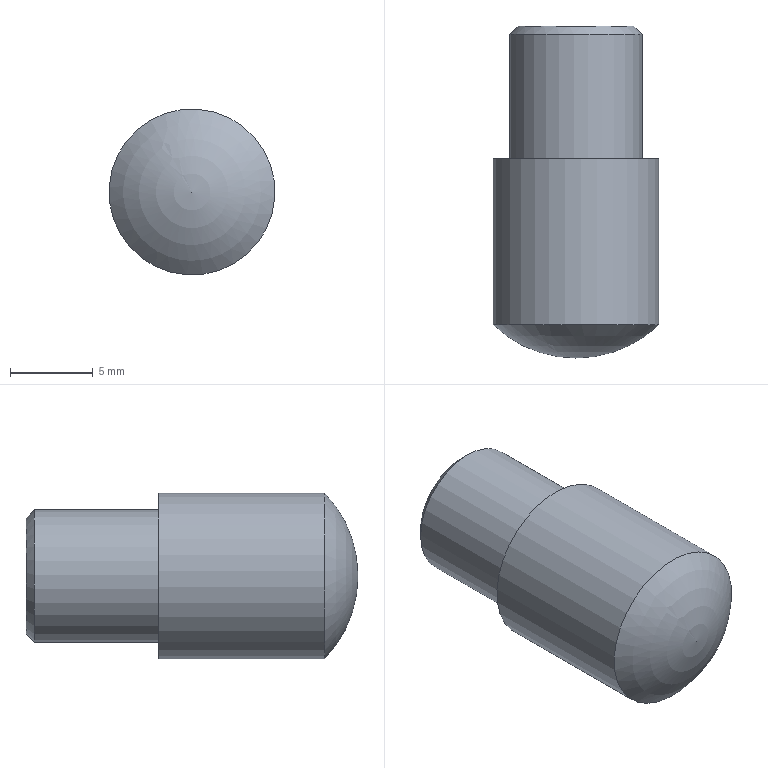Component | NX | 4_PIN | 1 solid | 6 faces | box 10 x 20 x 10 mm | volume 1267 mm3 | cylinder 2 | plane 2 | cone 1 | sphere 1 | commonest cylinder face diameters 10 x1 8 x1
STEP:
#1=CARTESIAN_POINT('',(0.,0.,0.));
#2=DIRECTION('',(0.,0.,1.));
#3=DIRECTION('',(1.,0.,0.));
#4=AXIS2_PLACEMENT_3D('',#1,#2,#3);
#5=CARTESIAN_POINT('',(6.35,16.63,-4.828));
#6=VERTEX_POINT('',#5);
#7=CARTESIAN_POINT('',(2.02,16.63,-7.328));
#8=DIRECTION('',(0.,-1.,0.));
#9=DIRECTION('',(0.866,0.,0.5));
#10=AXIS2_PLACEMENT_3D('',#7,#8,#9);
#11=CIRCLE('',#10,5.);
#12=CARTESIAN_POINT('',(2.02,4.63,-7.328));
#13=DIRECTION('',(0.,1.,0.));
#14=DIRECTION('',(0.866,0.,0.5));
#15=AXIS2_PLACEMENT_3D('',#12,#13,#14);
#16=CYLINDRICAL_SURFACE('',#15,5.);
#17=CARTESIAN_POINT('',(6.283,12.));
#18=DIRECTION('',(-1.,0.));
#19=VECTOR('',#18,1.);
#20=LINE('',#17,#19);
#21=(GEOMETRIC_REPRESENTATION_CONTEXT(2)PARAMETRIC_REPRESENTATION_CONTEXT()REPRESENTATION_CONTEXT('',''));
#22=DEFINITIONAL_REPRESENTATION('',(#20),#21);
#23=PCURVE('',#16,#22);
#24=CARTESIAN_POINT('',(2.02,16.63,-7.328));
#25=DIRECTION('',(0.,1.,0.));
#26=DIRECTION('',(0.866,0.,0.5));
#27=AXIS2_PLACEMENT_3D('',#24,#25,#26);
#28=PLANE('',#27);
#29=CARTESIAN_POINT('',(5.,0.));
#30=CARTESIAN_POINT('',(5.,-8.66));
#31=CARTESIAN_POINT('',(-2.5,-4.33));
#32=CARTESIAN_POINT('',(-10.,-0.));
#33=CARTESIAN_POINT('',(-2.5,4.33));
#34=CARTESIAN_POINT('',(5.,8.66));
#35=CARTESIAN_POINT('',(5.,0.));
#36=(BOUNDED_CURVE()B_SPLINE_CURVE(2,(#29,#30,#31,#32,#33,#34,#35),.UNSPECIFIED.,.T.,.F.)B_SPLINE_CURVE_WITH_KNOTS((1,2,2,2,2,1),(-2.094,0.,2.094,4.189,6.283,8.378),.UNSPECIFIED.)CURVE()GEOMETRIC_REPRESENTATION_ITEM()RATIONAL_B_SPLINE_CURVE((1.,0.5,1.,0.5,1.,0.5,1.))REPRESENTATION_ITEM(''));
#37=(GEOMETRIC_REPRESENTATION_CONTEXT(2)PARAMETRIC_REPRESENTATION_CONTEXT()REPRESENTATION_CONTEXT('',''));
#38=DEFINITIONAL_REPRESENTATION('',(#36),#37);
#39=PCURVE('',#28,#38);
#40=SURFACE_CURVE('',#11,(#23,#39),.PCURVE_S1.);
#41=EDGE_CURVE('',#6,#6,#40,.T.);
#42=ORIENTED_EDGE('',*,*,#41,.T.);
#43=CARTESIAN_POINT('',(6.35,6.63,-4.828));
#44=VERTEX_POINT('',#43);
#45=CARTESIAN_POINT('',(6.35,6.63,-4.828));
#46=CARTESIAN_POINT('',(6.35,16.63,-4.828));
#47=B_SPLINE_CURVE_WITH_KNOTS('',1,(#45,#46),.UNSPECIFIED.,.F.,.F.,(2,2),(2.,12.),.PIECEWISE_BEZIER_KNOTS.);
#48=CARTESIAN_POINT('',(0.,0.));
#49=DIRECTION('',(0.,1.));
#50=VECTOR('',#49,1.);
#51=LINE('',#48,#50);
#52=(GEOMETRIC_REPRESENTATION_CONTEXT(2)PARAMETRIC_REPRESENTATION_CONTEXT()REPRESENTATION_CONTEXT('',''));
#53=DEFINITIONAL_REPRESENTATION('',(#51),#52);
#54=PCURVE('',#16,#53);
#55=CARTESIAN_POINT('',(6.283,0.));
#56=DIRECTION('',(0.,1.));
#57=VECTOR('',#56,1.);
#58=LINE('',#55,#57);
#59=(GEOMETRIC_REPRESENTATION_CONTEXT(2)PARAMETRIC_REPRESENTATION_CONTEXT()REPRESENTATION_CONTEXT('',''));
#60=DEFINITIONAL_REPRESENTATION('',(#58),#59);
#61=PCURVE('',#16,#60);
#62=SEAM_CURVE('',#47,(#54,#61),.PCURVE_S1.);
#63=EDGE_CURVE('',#44,#6,#62,.T.);
#64=ORIENTED_EDGE('',*,*,#63,.F.);
#65=CARTESIAN_POINT('',(-0.4796,6.63,-2.998));
#66=VERTEX_POINT('',#65);
#67=CARTESIAN_POINT('',(2.02,6.63,-7.328));
#68=DIRECTION('',(0.,1.,0.));
#69=DIRECTION('',(0.866,0.,0.5));
#70=AXIS2_PLACEMENT_3D('',#67,#68,#69);
#71=CIRCLE('',#70,5.);
#72=CARTESIAN_POINT('',(0.,2.));
#73=DIRECTION('',(1.,0.));
#74=VECTOR('',#73,1.);
#75=LINE('',#72,#74);
#76=(GEOMETRIC_REPRESENTATION_CONTEXT(2)PARAMETRIC_REPRESENTATION_CONTEXT()REPRESENTATION_CONTEXT('',''));
#77=DEFINITIONAL_REPRESENTATION('',(#75),#76);
#78=PCURVE('',#16,#77);
#79=CARTESIAN_POINT('',(2.02,11.88,-7.328));
#80=DIRECTION('',(-0.,1.,0.));
#81=DIRECTION('',(-0.5,-0.,0.866));
#82=AXIS2_PLACEMENT_3D('',#79,#80,#81);
#83=SPHERICAL_SURFACE('',#82,7.25);
#84=CARTESIAN_POINT('',(1.571,-0.8098));
#85=CARTESIAN_POINT('',(1.666,-0.8098));
#86=CARTESIAN_POINT('',(1.856,-0.8098));
#87=CARTESIAN_POINT('',(2.142,-0.8098));
#88=CARTESIAN_POINT('',(2.428,-0.8098));
#89=CARTESIAN_POINT('',(2.713,-0.8098));
#90=CARTESIAN_POINT('',(2.999,-0.8098));
#91=CARTESIAN_POINT('',(3.284,-0.8098));
#92=CARTESIAN_POINT('',(3.57,-0.8098));
#93=CARTESIAN_POINT('',(3.856,-0.8098));
#94=CARTESIAN_POINT('',(4.141,-0.8098));
#95=CARTESIAN_POINT('',(4.427,-0.8098));
#96=CARTESIAN_POINT('',(4.712,-0.8098));
#97=CARTESIAN_POINT('',(4.998,-0.8098));
#98=CARTESIAN_POINT('',(5.284,-0.8098));
#99=CARTESIAN_POINT('',(5.569,-0.8098));
#100=CARTESIAN_POINT('',(5.855,-0.8098));
#101=CARTESIAN_POINT('',(6.14,-0.8098));
#102=CARTESIAN_POINT('',(6.426,-0.8098));
#103=CARTESIAN_POINT('',(6.712,-0.8098));
#104=CARTESIAN_POINT('',(6.997,-0.8098));
#105=CARTESIAN_POINT('',(7.283,-0.8098));
#106=CARTESIAN_POINT('',(7.568,-0.8098));
#107=CARTESIAN_POINT('',(7.759,-0.8098));
#108=CARTESIAN_POINT('',(7.854,-0.8098));
#109=B_SPLINE_CURVE_WITH_KNOTS('',3,(#84,#85,#86,#87,#88,#89,#90,#91,#92,#93,#94,#95,#96,#97,#98,#99,#100,#101,#102,#103,#104,#105,#106,#107,#108),.UNSPECIFIED.,.F.,.F.,(4,1,1,1,1,1,1,1,1,1,1,1,1,1,1,1,1,1,1,1,1,1,4),(0.,0.2856,0.5712,0.8568,1.142,1.428,1.714,1.999,2.285,2.57,2.856,3.142,3.427,3.713,3.998,4.284,4.57,4.855,5.141,5.426,5.712,5.998,6.283),.QUASI_UNIFORM_KNOTS.);
#110=(GEOMETRIC_REPRESENTATION_CONTEXT(2)PARAMETRIC_REPRESENTATION_CONTEXT()REPRESENTATION_CONTEXT('',''));
#111=DEFINITIONAL_REPRESENTATION('',(#109),#110);
#112=PCURVE('',#83,#111);
#113=SURFACE_CURVE('',#71,(#78,#112),.PCURVE_S1.);
#114=EDGE_CURVE('',#44,#66,#113,.T.);
#115=ORIENTED_EDGE('',*,*,#114,.T.);
#116=CARTESIAN_POINT('',(2.02,6.63,-7.328));
#117=DIRECTION('',(0.,1.,0.));
#118=DIRECTION('',(0.866,0.,0.5));
#119=AXIS2_PLACEMENT_3D('',#116,#117,#118);
#120=CIRCLE('',#119,5.);
#121=CARTESIAN_POINT('',(0.,2.));
#122=DIRECTION('',(1.,0.));
#123=VECTOR('',#122,1.);
#124=LINE('',#121,#123);
#125=(GEOMETRIC_REPRESENTATION_CONTEXT(2)PARAMETRIC_REPRESENTATION_CONTEXT()REPRESENTATION_CONTEXT('',''));
#126=DEFINITIONAL_REPRESENTATION('',(#124),#125);
#127=PCURVE('',#16,#126);
#128=CARTESIAN_POINT('',(-4.712,-0.8098));
#129=CARTESIAN_POINT('',(-4.617,-0.8098));
#130=CARTESIAN_POINT('',(-4.427,-0.8098));
#131=CARTESIAN_POINT('',(-4.141,-0.8098));
#132=CARTESIAN_POINT('',(-3.856,-0.8098));
#133=CARTESIAN_POINT('',(-3.57,-0.8098));
#134=CARTESIAN_POINT('',(-3.284,-0.8098));
#135=CARTESIAN_POINT('',(-2.999,-0.8098));
#136=CARTESIAN_POINT('',(-2.713,-0.8098));
#137=CARTESIAN_POINT('',(-2.428,-0.8098));
#138=CARTESIAN_POINT('',(-2.142,-0.8098));
#139=CARTESIAN_POINT('',(-1.856,-0.8098));
#140=CARTESIAN_POINT('',(-1.571,-0.8098));
#141=CARTESIAN_POINT('',(-1.285,-0.8098));
#142=CARTESIAN_POINT('',(-0.9996,-0.8098));
#143=CARTESIAN_POINT('',(-0.714,-0.8098));
#144=CARTESIAN_POINT('',(-0.4284,-0.8098));
#145=CARTESIAN_POINT('',(-0.1428,-0.8098));
#146=CARTESIAN_POINT('',(0.1428,-0.8098));
#147=CARTESIAN_POINT('',(0.4284,-0.8098));
#148=CARTESIAN_POINT('',(0.714,-0.8098));
#149=CARTESIAN_POINT('',(0.9996,-0.8098));
#150=CARTESIAN_POINT('',(1.285,-0.8098));
#151=CARTESIAN_POINT('',(1.476,-0.8098));
#152=CARTESIAN_POINT('',(1.571,-0.8098));
#153=B_SPLINE_CURVE_WITH_KNOTS('',3,(#128,#129,#130,#131,#132,#133,#134,#135,#136,#137,#138,#139,#140,#141,#142,#143,#144,#145,#146,#147,#148,#149,#150,#151,#152),.UNSPECIFIED.,.F.,.F.,(4,1,1,1,1,1,1,1,1,1,1,1,1,1,1,1,1,1,1,1,1,1,4),(0.,0.2856,0.5712,0.8568,1.142,1.428,1.714,1.999,2.285,2.57,2.856,3.142,3.427,3.713,3.998,4.284,4.57,4.855,5.141,5.426,5.712,5.998,6.283),.QUASI_UNIFORM_KNOTS.);
#154=(GEOMETRIC_REPRESENTATION_CONTEXT(2)PARAMETRIC_REPRESENTATION_CONTEXT()REPRESENTATION_CONTEXT('',''));
#155=DEFINITIONAL_REPRESENTATION('',(#153),#154);
#156=PCURVE('',#83,#155);
#157=SURFACE_CURVE('',#120,(#127,#156),.PCURVE_S1.);
#158=EDGE_CURVE('',#66,#44,#157,.T.);
#159=ORIENTED_EDGE('',*,*,#158,.T.);
#160=ORIENTED_EDGE('',*,*,#63,.T.);
#161=EDGE_LOOP('',(#42,#64,#115,#159,#160));
#162=FACE_BOUND('',#161,.T.);
#163=ADVANCED_FACE('',(#162),#16,.T.);
#164=CARTESIAN_POINT('',(5.484,16.63,-5.328));
#165=VERTEX_POINT('',#164);
#166=CARTESIAN_POINT('',(2.02,16.63,-7.328));
#167=DIRECTION('',(0.,1.,0.));
#168=DIRECTION('',(0.866,0.,0.5));
#169=AXIS2_PLACEMENT_3D('',#166,#167,#168);
#170=CIRCLE('',#169,4.);
#171=CARTESIAN_POINT('',(0.,0.));
#172=DIRECTION('',(1.,0.));
#173=AXIS2_PLACEMENT_2D('',#171,#172);
#174=CIRCLE('',#173,4.);
#175=(GEOMETRIC_REPRESENTATION_CONTEXT(2)PARAMETRIC_REPRESENTATION_CONTEXT()REPRESENTATION_CONTEXT('',''));
#176=DEFINITIONAL_REPRESENTATION('',(#174),#175);
#177=PCURVE('',#28,#176);
#178=CARTESIAN_POINT('',(2.02,16.63,-7.328));
#179=DIRECTION('',(0.,1.,0.));
#180=DIRECTION('',(0.866,0.,0.5));
#181=AXIS2_PLACEMENT_3D('',#178,#179,#180);
#182=CYLINDRICAL_SURFACE('',#181,4.);
#183=CARTESIAN_POINT('',(0.,0.));
#184=DIRECTION('',(1.,0.));
#185=VECTOR('',#184,1.);
#186=LINE('',#183,#185);
#187=(GEOMETRIC_REPRESENTATION_CONTEXT(2)PARAMETRIC_REPRESENTATION_CONTEXT()REPRESENTATION_CONTEXT('',''));
#188=DEFINITIONAL_REPRESENTATION('',(#186),#187);
#189=PCURVE('',#182,#188);
#190=SURFACE_CURVE('',#170,(#177,#189),.PCURVE_S1.);
#191=EDGE_CURVE('',#165,#165,#190,.T.);
#192=ORIENTED_EDGE('',*,*,#191,.F.);
#193=EDGE_LOOP('',(#192));
#194=FACE_BOUND('',#193,.T.);
#195=ORIENTED_EDGE('',*,*,#41,.F.);
#196=EDGE_LOOP('',(#195));
#197=FACE_BOUND('',#196,.T.);
#198=ADVANCED_FACE('',(#194,#197),#28,.T.);
#199=CARTESIAN_POINT('',(5.051,24.63,-5.578));
#200=VERTEX_POINT('',#199);
#201=CARTESIAN_POINT('',(2.02,24.63,-7.328));
#202=DIRECTION('',(0.,1.,0.));
#203=DIRECTION('',(0.866,0.,0.5));
#204=AXIS2_PLACEMENT_3D('',#201,#202,#203);
#205=CIRCLE('',#204,3.5);
#206=CARTESIAN_POINT('',(2.02,24.63,-7.328));
#207=DIRECTION('',(0.,1.,0.));
#208=DIRECTION('',(0.866,0.,0.5));
#209=AXIS2_PLACEMENT_3D('',#206,#207,#208);
#210=PLANE('',#209);
#211=CARTESIAN_POINT('',(0.,0.));
#212=DIRECTION('',(1.,0.));
#213=AXIS2_PLACEMENT_2D('',#211,#212);
#214=CIRCLE('',#213,3.5);
#215=(GEOMETRIC_REPRESENTATION_CONTEXT(2)PARAMETRIC_REPRESENTATION_CONTEXT()REPRESENTATION_CONTEXT('',''));
#216=DEFINITIONAL_REPRESENTATION('',(#214),#215);
#217=PCURVE('',#210,#216);
#218=CARTESIAN_POINT('',(2.02,24.13,-7.328));
#219=DIRECTION('',(0.,-1.,0.));
#220=DIRECTION('',(-0.866,0.,-0.5));
#221=AXIS2_PLACEMENT_3D('',#218,#219,#220);
#222=CONICAL_SURFACE('',#221,4.,0.7854);
#223=CARTESIAN_POINT('',(9.425,-0.5));
#224=DIRECTION('',(-1.,-0.));
#225=VECTOR('',#224,1.);
#226=LINE('',#223,#225);
#227=(GEOMETRIC_REPRESENTATION_CONTEXT(2)PARAMETRIC_REPRESENTATION_CONTEXT()REPRESENTATION_CONTEXT('',''));
#228=DEFINITIONAL_REPRESENTATION('',(#226),#227);
#229=PCURVE('',#222,#228);
#230=SURFACE_CURVE('',#205,(#217,#229),.PCURVE_S1.);
#231=EDGE_CURVE('',#200,#200,#230,.T.);
#232=ORIENTED_EDGE('',*,*,#231,.T.);
#233=EDGE_LOOP('',(#232));
#234=FACE_BOUND('',#233,.T.);
#235=ADVANCED_FACE('',(#234),#210,.T.);
#236=CARTESIAN_POINT('',(5.484,24.13,-5.328));
#237=VERTEX_POINT('',#236);
#238=CARTESIAN_POINT('',(2.02,24.13,-7.328));
#239=DIRECTION('',(0.,-1.,0.));
#240=DIRECTION('',(0.866,0.,0.5));
#241=AXIS2_PLACEMENT_3D('',#238,#239,#240);
#242=CIRCLE('',#241,4.);
#243=CARTESIAN_POINT('',(6.283,7.5));
#244=DIRECTION('',(-1.,0.));
#245=VECTOR('',#244,1.);
#246=LINE('',#243,#245);
#247=(GEOMETRIC_REPRESENTATION_CONTEXT(2)PARAMETRIC_REPRESENTATION_CONTEXT()REPRESENTATION_CONTEXT('',''));
#248=DEFINITIONAL_REPRESENTATION('',(#246),#247);
#249=PCURVE('',#182,#248);
#250=CARTESIAN_POINT('',(3.142,0.));
#251=DIRECTION('',(1.,0.));
#252=VECTOR('',#251,1.);
#253=LINE('',#250,#252);
#254=(GEOMETRIC_REPRESENTATION_CONTEXT(2)PARAMETRIC_REPRESENTATION_CONTEXT()REPRESENTATION_CONTEXT('',''));
#255=DEFINITIONAL_REPRESENTATION('',(#253),#254);
#256=PCURVE('',#222,#255);
#257=SURFACE_CURVE('',#242,(#249,#256),.PCURVE_S1.);
#258=EDGE_CURVE('',#237,#237,#257,.T.);
#259=ORIENTED_EDGE('',*,*,#258,.T.);
#260=CARTESIAN_POINT('',(5.484,16.63,-5.328));
#261=CARTESIAN_POINT('',(5.484,24.13,-5.328));
#262=B_SPLINE_CURVE_WITH_KNOTS('',1,(#260,#261),.UNSPECIFIED.,.F.,.F.,(2,2),(0.,7.5),.PIECEWISE_BEZIER_KNOTS.);
#263=CARTESIAN_POINT('',(0.,0.));
#264=DIRECTION('',(0.,1.));
#265=VECTOR('',#264,1.);
#266=LINE('',#263,#265);
#267=(GEOMETRIC_REPRESENTATION_CONTEXT(2)PARAMETRIC_REPRESENTATION_CONTEXT()REPRESENTATION_CONTEXT('',''));
#268=DEFINITIONAL_REPRESENTATION('',(#266),#267);
#269=PCURVE('',#182,#268);
#270=CARTESIAN_POINT('',(6.283,0.));
#271=DIRECTION('',(0.,1.));
#272=VECTOR('',#271,1.);
#273=LINE('',#270,#272);
#274=(GEOMETRIC_REPRESENTATION_CONTEXT(2)PARAMETRIC_REPRESENTATION_CONTEXT()REPRESENTATION_CONTEXT('',''));
#275=DEFINITIONAL_REPRESENTATION('',(#273),#274);
#276=PCURVE('',#182,#275);
#277=SEAM_CURVE('',#262,(#269,#276),.PCURVE_S1.);
#278=EDGE_CURVE('',#165,#237,#277,.T.);
#279=ORIENTED_EDGE('',*,*,#278,.F.);
#280=ORIENTED_EDGE('',*,*,#191,.T.);
#281=ORIENTED_EDGE('',*,*,#278,.T.);
#282=EDGE_LOOP('',(#259,#279,#280,#281));
#283=FACE_BOUND('',#282,.T.);
#284=ADVANCED_FACE('',(#283),#182,.T.);
#285=ORIENTED_EDGE('',*,*,#231,.F.);
#286=CARTESIAN_POINT('',(5.051,24.63,-5.578));
#287=CARTESIAN_POINT('',(5.484,24.13,-5.328));
#288=B_SPLINE_CURVE_WITH_KNOTS('',1,(#286,#287),.UNSPECIFIED.,.F.,.F.,(2,2),(-0.7071,0.),.PIECEWISE_BEZIER_KNOTS.);
#289=CARTESIAN_POINT('',(9.425,0.));
#290=DIRECTION('',(0.,1.));
#291=VECTOR('',#290,1.);
#292=LINE('',#289,#291);
#293=(GEOMETRIC_REPRESENTATION_CONTEXT(2)PARAMETRIC_REPRESENTATION_CONTEXT()REPRESENTATION_CONTEXT('',''));
#294=DEFINITIONAL_REPRESENTATION('',(#292),#293);
#295=PCURVE('',#222,#294);
#296=CARTESIAN_POINT('',(3.142,0.));
#297=DIRECTION('',(0.,1.));
#298=VECTOR('',#297,1.);
#299=LINE('',#296,#298);
#300=(GEOMETRIC_REPRESENTATION_CONTEXT(2)PARAMETRIC_REPRESENTATION_CONTEXT()REPRESENTATION_CONTEXT('',''));
#301=DEFINITIONAL_REPRESENTATION('',(#299),#300);
#302=PCURVE('',#222,#301);
#303=SEAM_CURVE('',#288,(#295,#302),.PCURVE_S1.);
#304=EDGE_CURVE('',#200,#237,#303,.T.);
#305=ORIENTED_EDGE('',*,*,#304,.T.);
#306=ORIENTED_EDGE('',*,*,#258,.F.);
#307=ORIENTED_EDGE('',*,*,#304,.F.);
#308=EDGE_LOOP('',(#285,#305,#306,#307));
#309=FACE_BOUND('',#308,.T.);
#310=ADVANCED_FACE('',(#309),#222,.T.);
#311=CARTESIAN_POINT('',(2.02,4.63,-7.328));
#312=VERTEX_POINT('',#311);
#313=CARTESIAN_POINT('',(2.02,4.63,-7.328));
#314=CARTESIAN_POINT('',(1.469,4.63,-6.372));
#315=CARTESIAN_POINT('',(0.9169,4.84,-5.417));
#316=CARTESIAN_POINT('',(0.3918,5.26,-4.507));
#317=CARTESIAN_POINT('',(-0.0801,5.869,-3.69));
#318=CARTESIAN_POINT('',(-0.4796,6.63,-2.998));
#319=B_SPLINE_CURVE_WITH_KNOTS('',5,(#313,#314,#315,#316,#317,#318),.UNSPECIFIED.,.F.,.F.,(6,6),(-1.571,-0.8098),.PIECEWISE_BEZIER_KNOTS.);
#320=CARTESIAN_POINT('',(6.283,0.));
#321=DIRECTION('',(0.,1.));
#322=VECTOR('',#321,1.);
#323=LINE('',#320,#322);
#324=(GEOMETRIC_REPRESENTATION_CONTEXT(2)PARAMETRIC_REPRESENTATION_CONTEXT()REPRESENTATION_CONTEXT('',''));
#325=DEFINITIONAL_REPRESENTATION('',(#323),#324);
#326=PCURVE('',#83,#325);
#327=CARTESIAN_POINT('',(0.,0.));
#328=DIRECTION('',(0.,1.));
#329=VECTOR('',#328,1.);
#330=LINE('',#327,#329);
#331=(GEOMETRIC_REPRESENTATION_CONTEXT(2)PARAMETRIC_REPRESENTATION_CONTEXT()REPRESENTATION_CONTEXT('',''));
#332=DEFINITIONAL_REPRESENTATION('',(#330),#331);
#333=PCURVE('',#83,#332);
#334=SEAM_CURVE('',#319,(#326,#333),.PCURVE_S1.);
#335=EDGE_CURVE('',#312,#66,#334,.T.);
#336=ORIENTED_EDGE('',*,*,#335,.T.);
#337=ORIENTED_EDGE('',*,*,#114,.F.);
#338=ORIENTED_EDGE('',*,*,#158,.F.);
#339=ORIENTED_EDGE('',*,*,#335,.F.);
#340=EDGE_LOOP('',(#336,#337,#338,#339));
#341=FACE_BOUND('',#340,.T.);
#342=ADVANCED_FACE('',(#341),#83,.T.);
#343=CLOSED_SHELL('',(#163,#198,#235,#284,#310,#342));
#344=MANIFOLD_SOLID_BREP('',#343);
#345=(LENGTH_UNIT()NAMED_UNIT(*)SI_UNIT(.MILLI.,.METRE.));
#346=UNCERTAINTY_MEASURE_WITH_UNIT(LENGTH_MEASURE(0.00001),#345,'','');
#347=(NAMED_UNIT(*)PLANE_ANGLE_UNIT()SI_UNIT($,.RADIAN.));
#348=(NAMED_UNIT(*)SI_UNIT($,.STERADIAN.)SOLID_ANGLE_UNIT());
#349=(GEOMETRIC_REPRESENTATION_CONTEXT(3)GLOBAL_UNCERTAINTY_ASSIGNED_CONTEXT((#346))GLOBAL_UNIT_ASSIGNED_CONTEXT((#345,#347,#348))REPRESENTATION_CONTEXT('',''));
#350=ADVANCED_BREP_SHAPE_REPRESENTATION('',(#4,#344),#349);